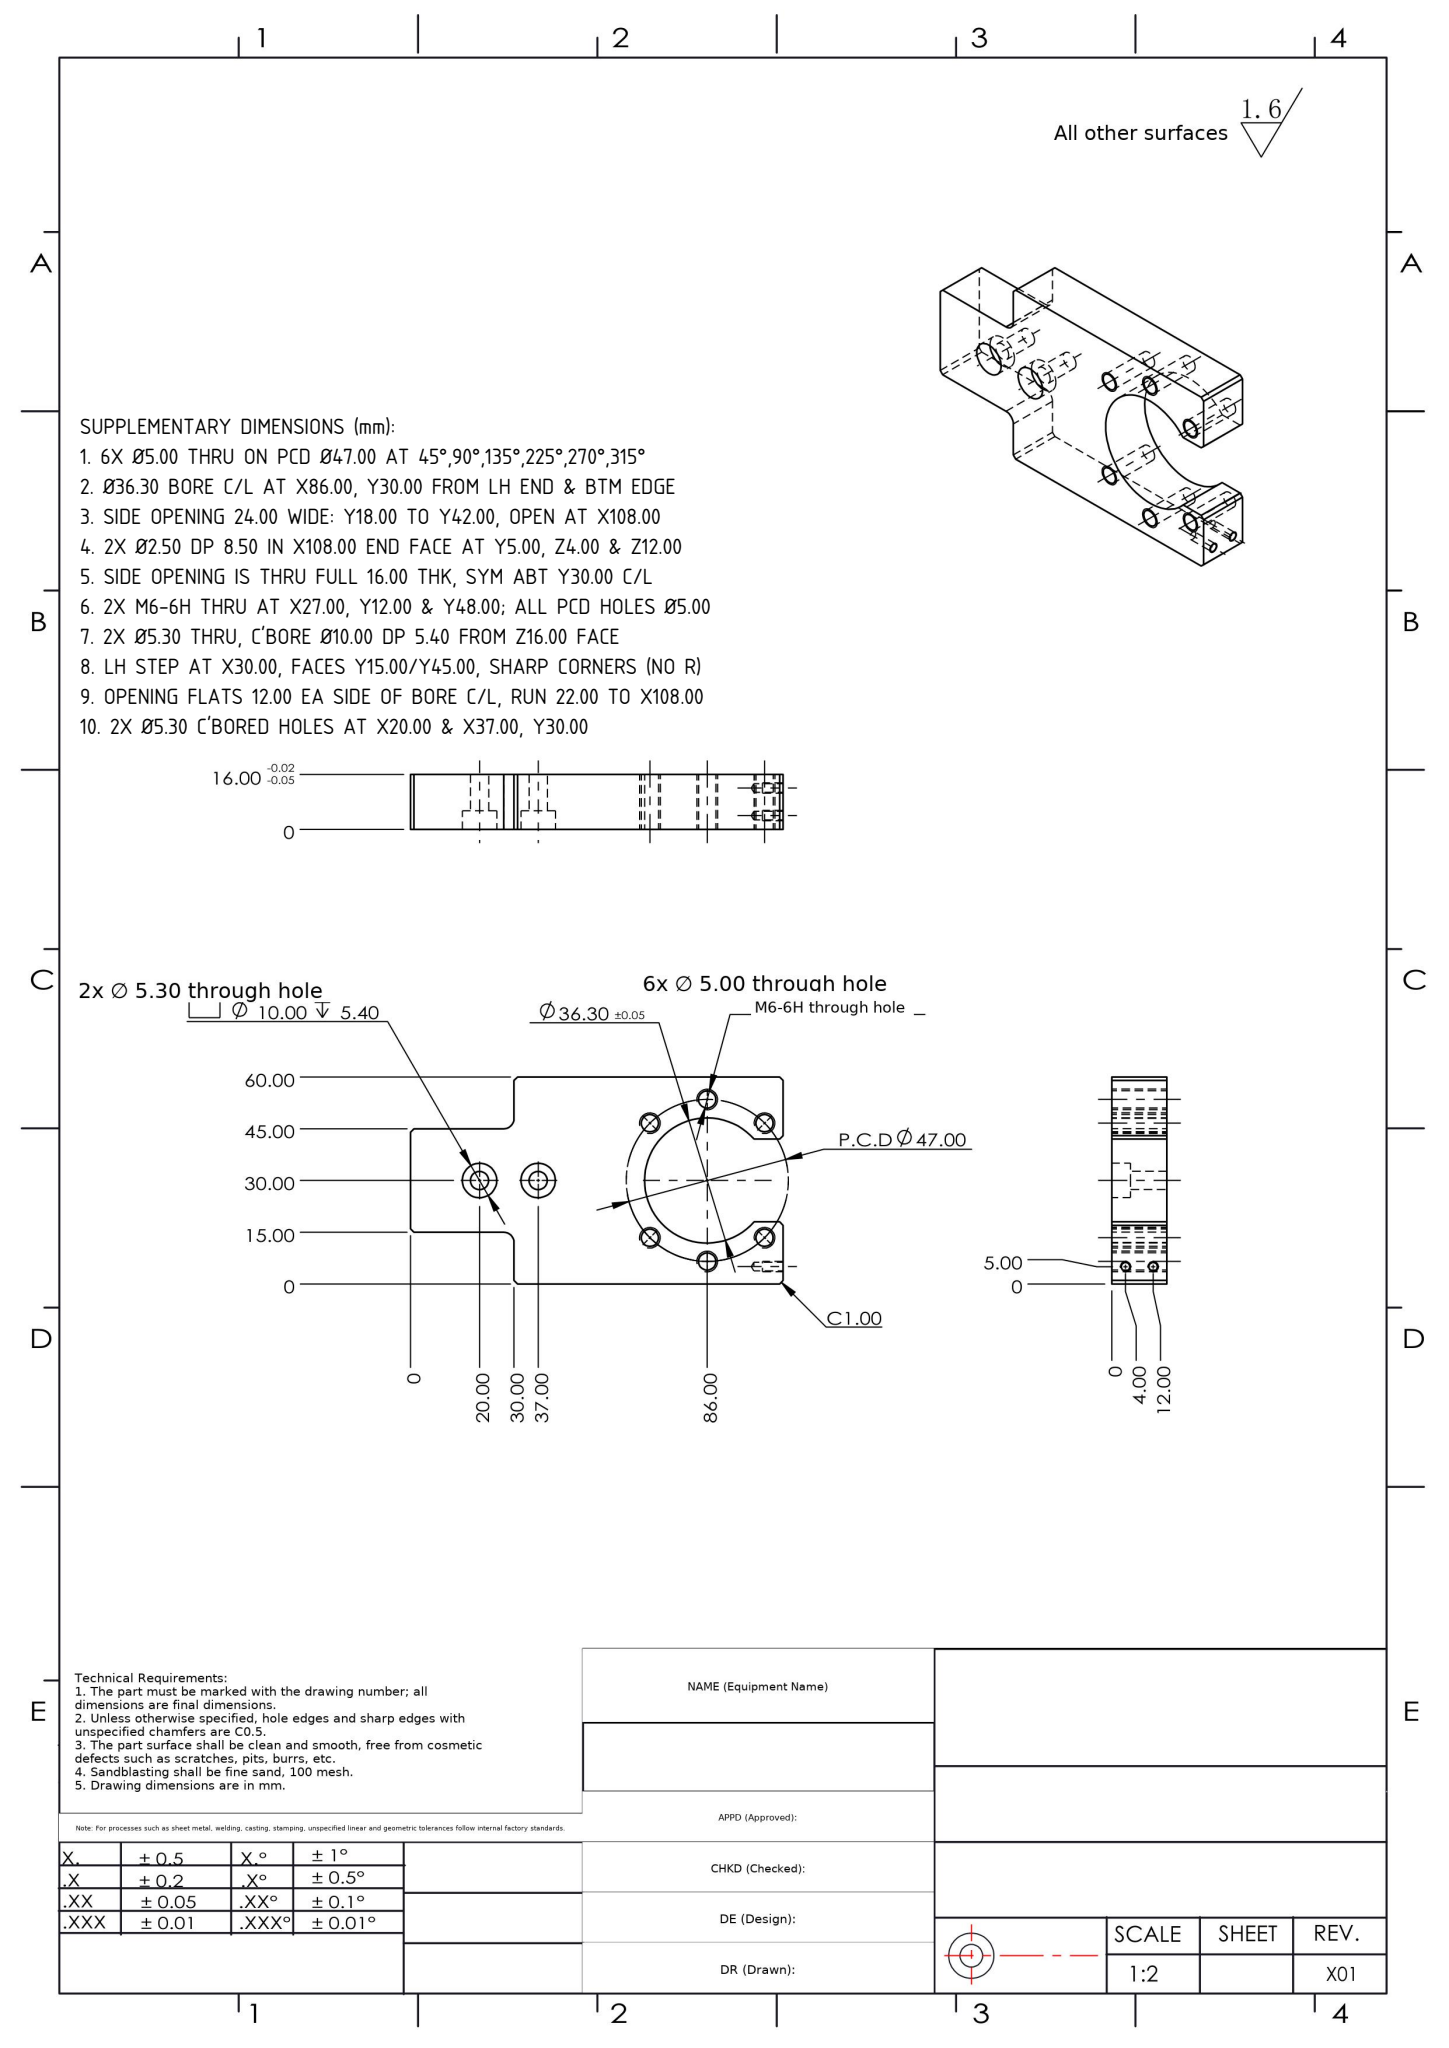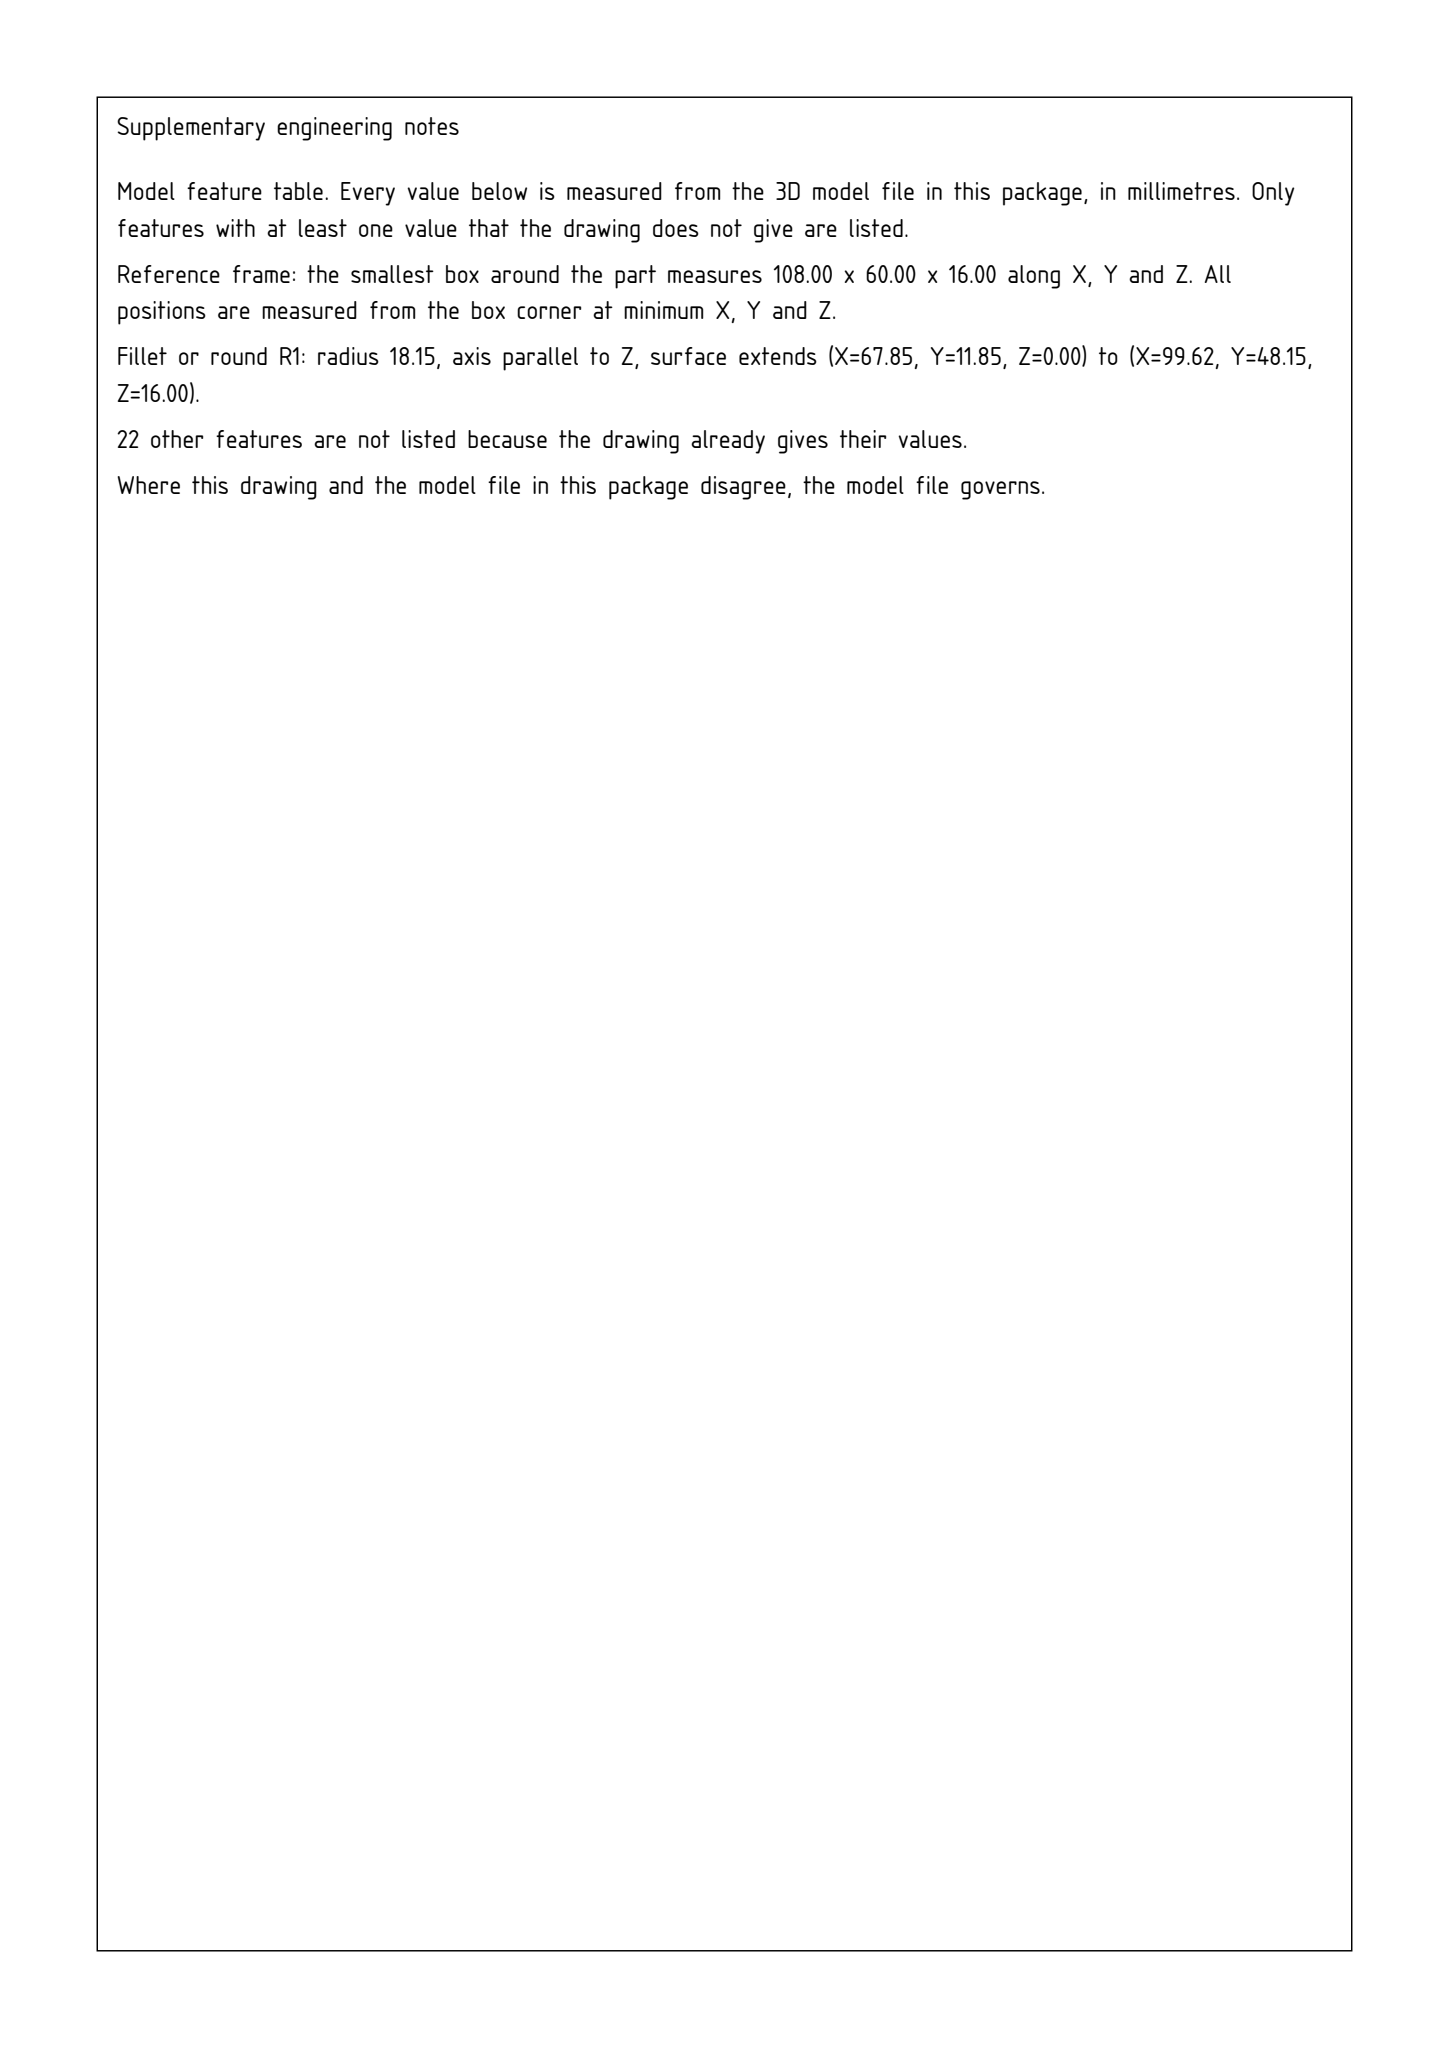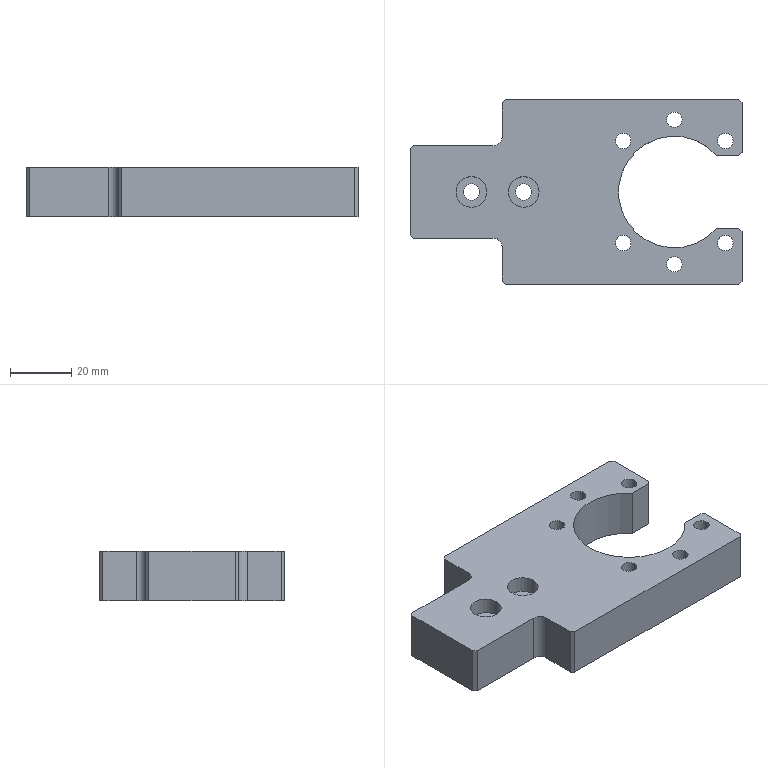Part | SolidWorks | mm | 1 solid | 54 faces | box 108 x 60 x 16 mm | volume 67406 mm3 | cylinder 27 | plane 23 | cone 4 | commonest cylinder face diameters 5 x12 2.5 x4 10 x4 5.3 x4 6 x2 36.3 x1